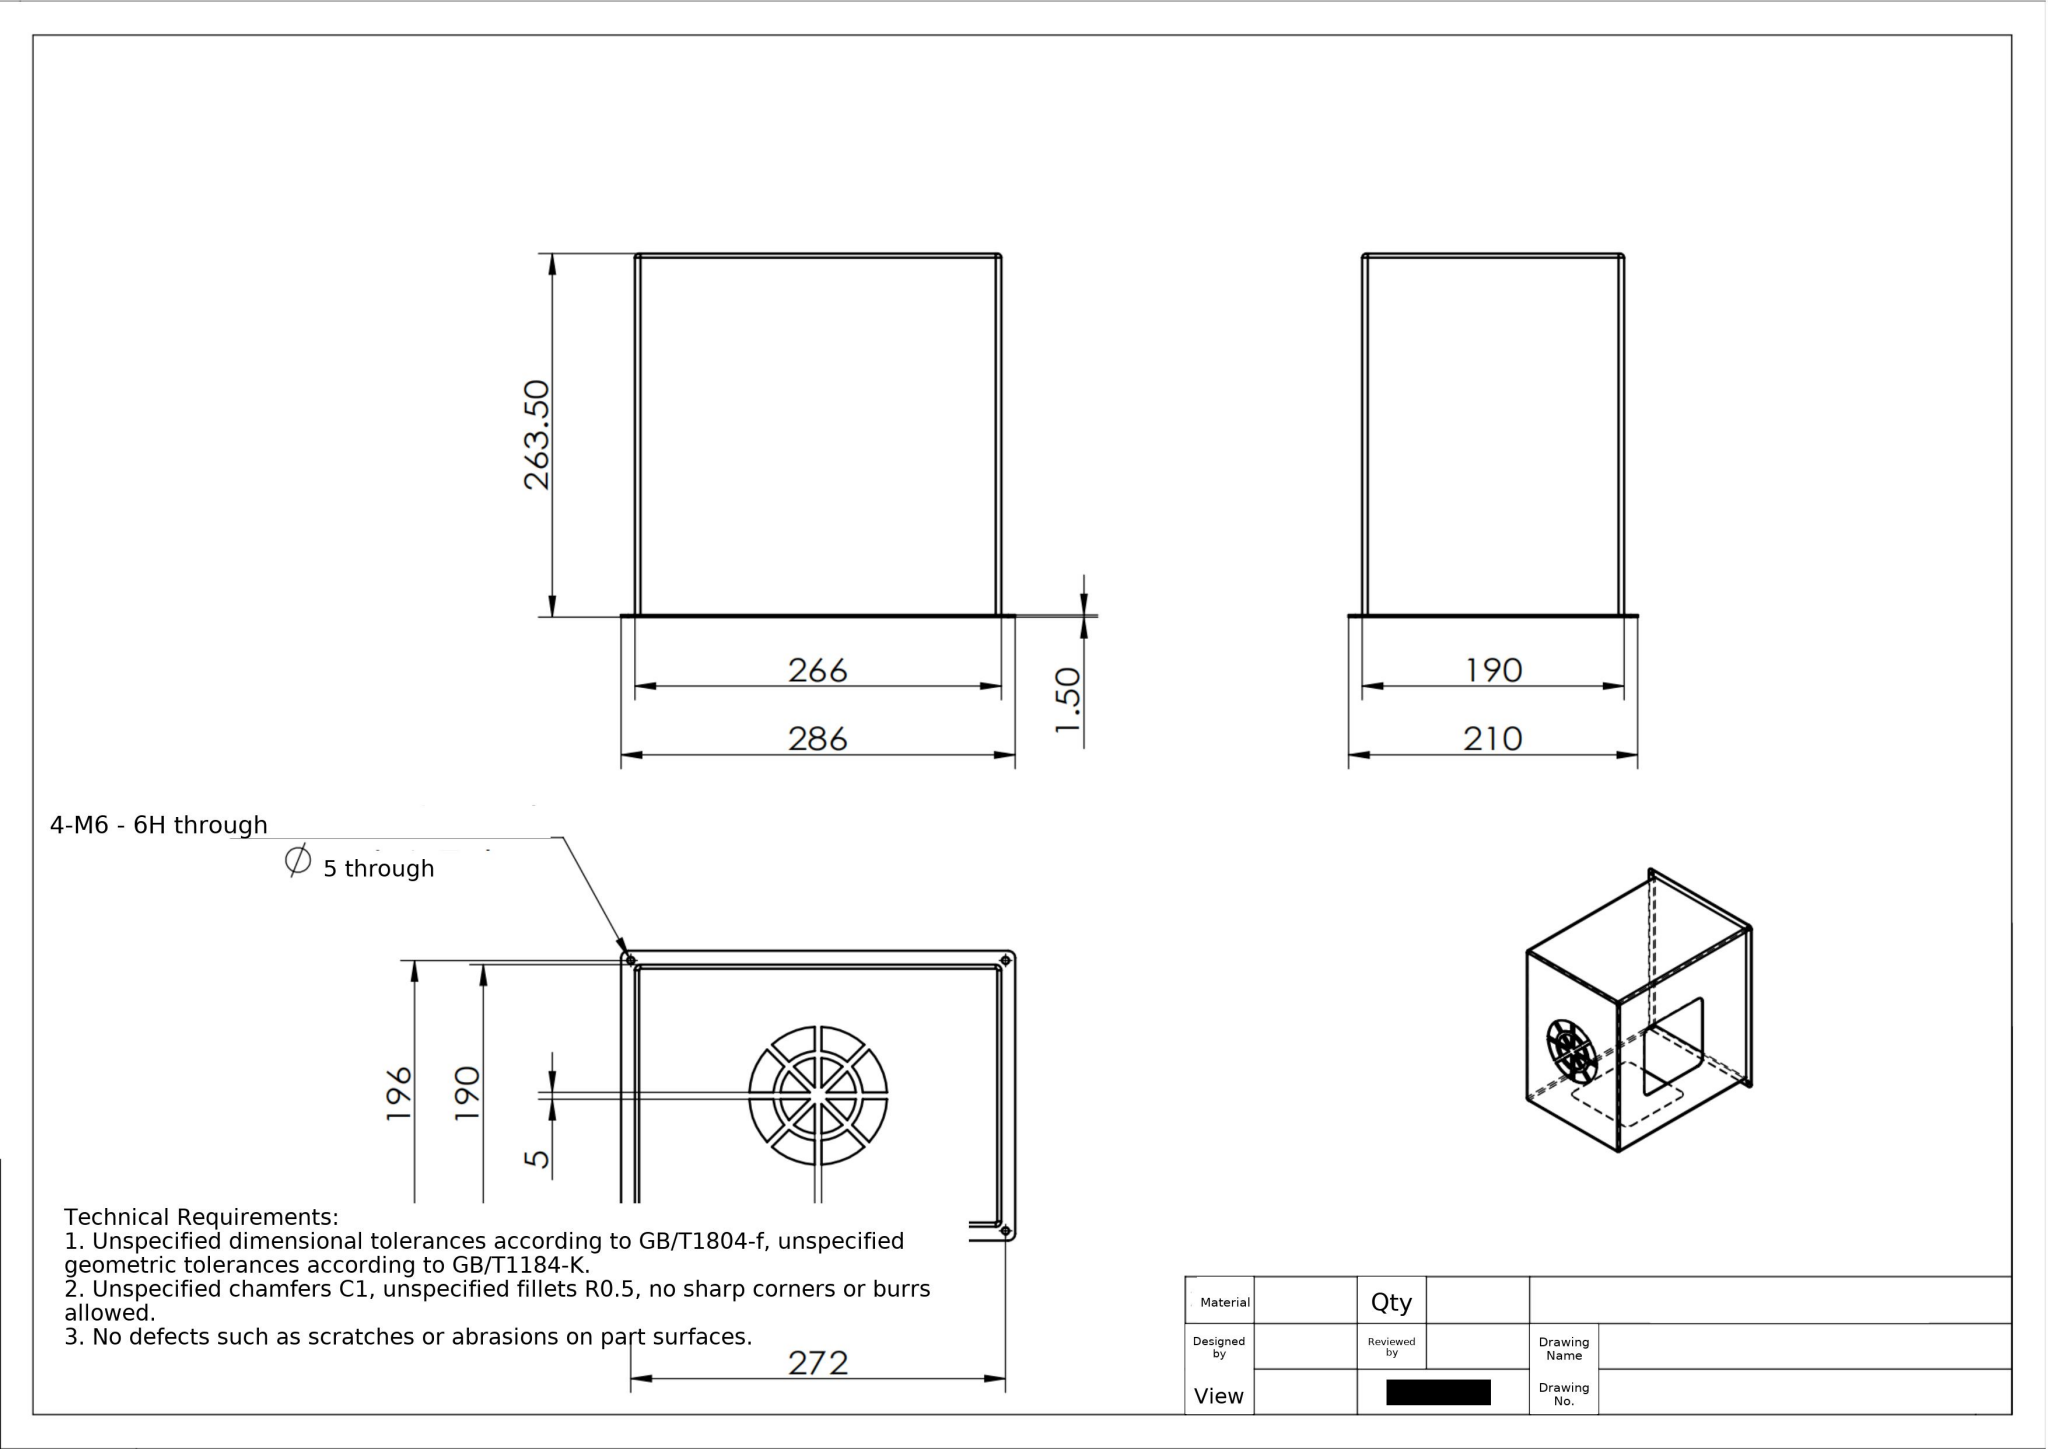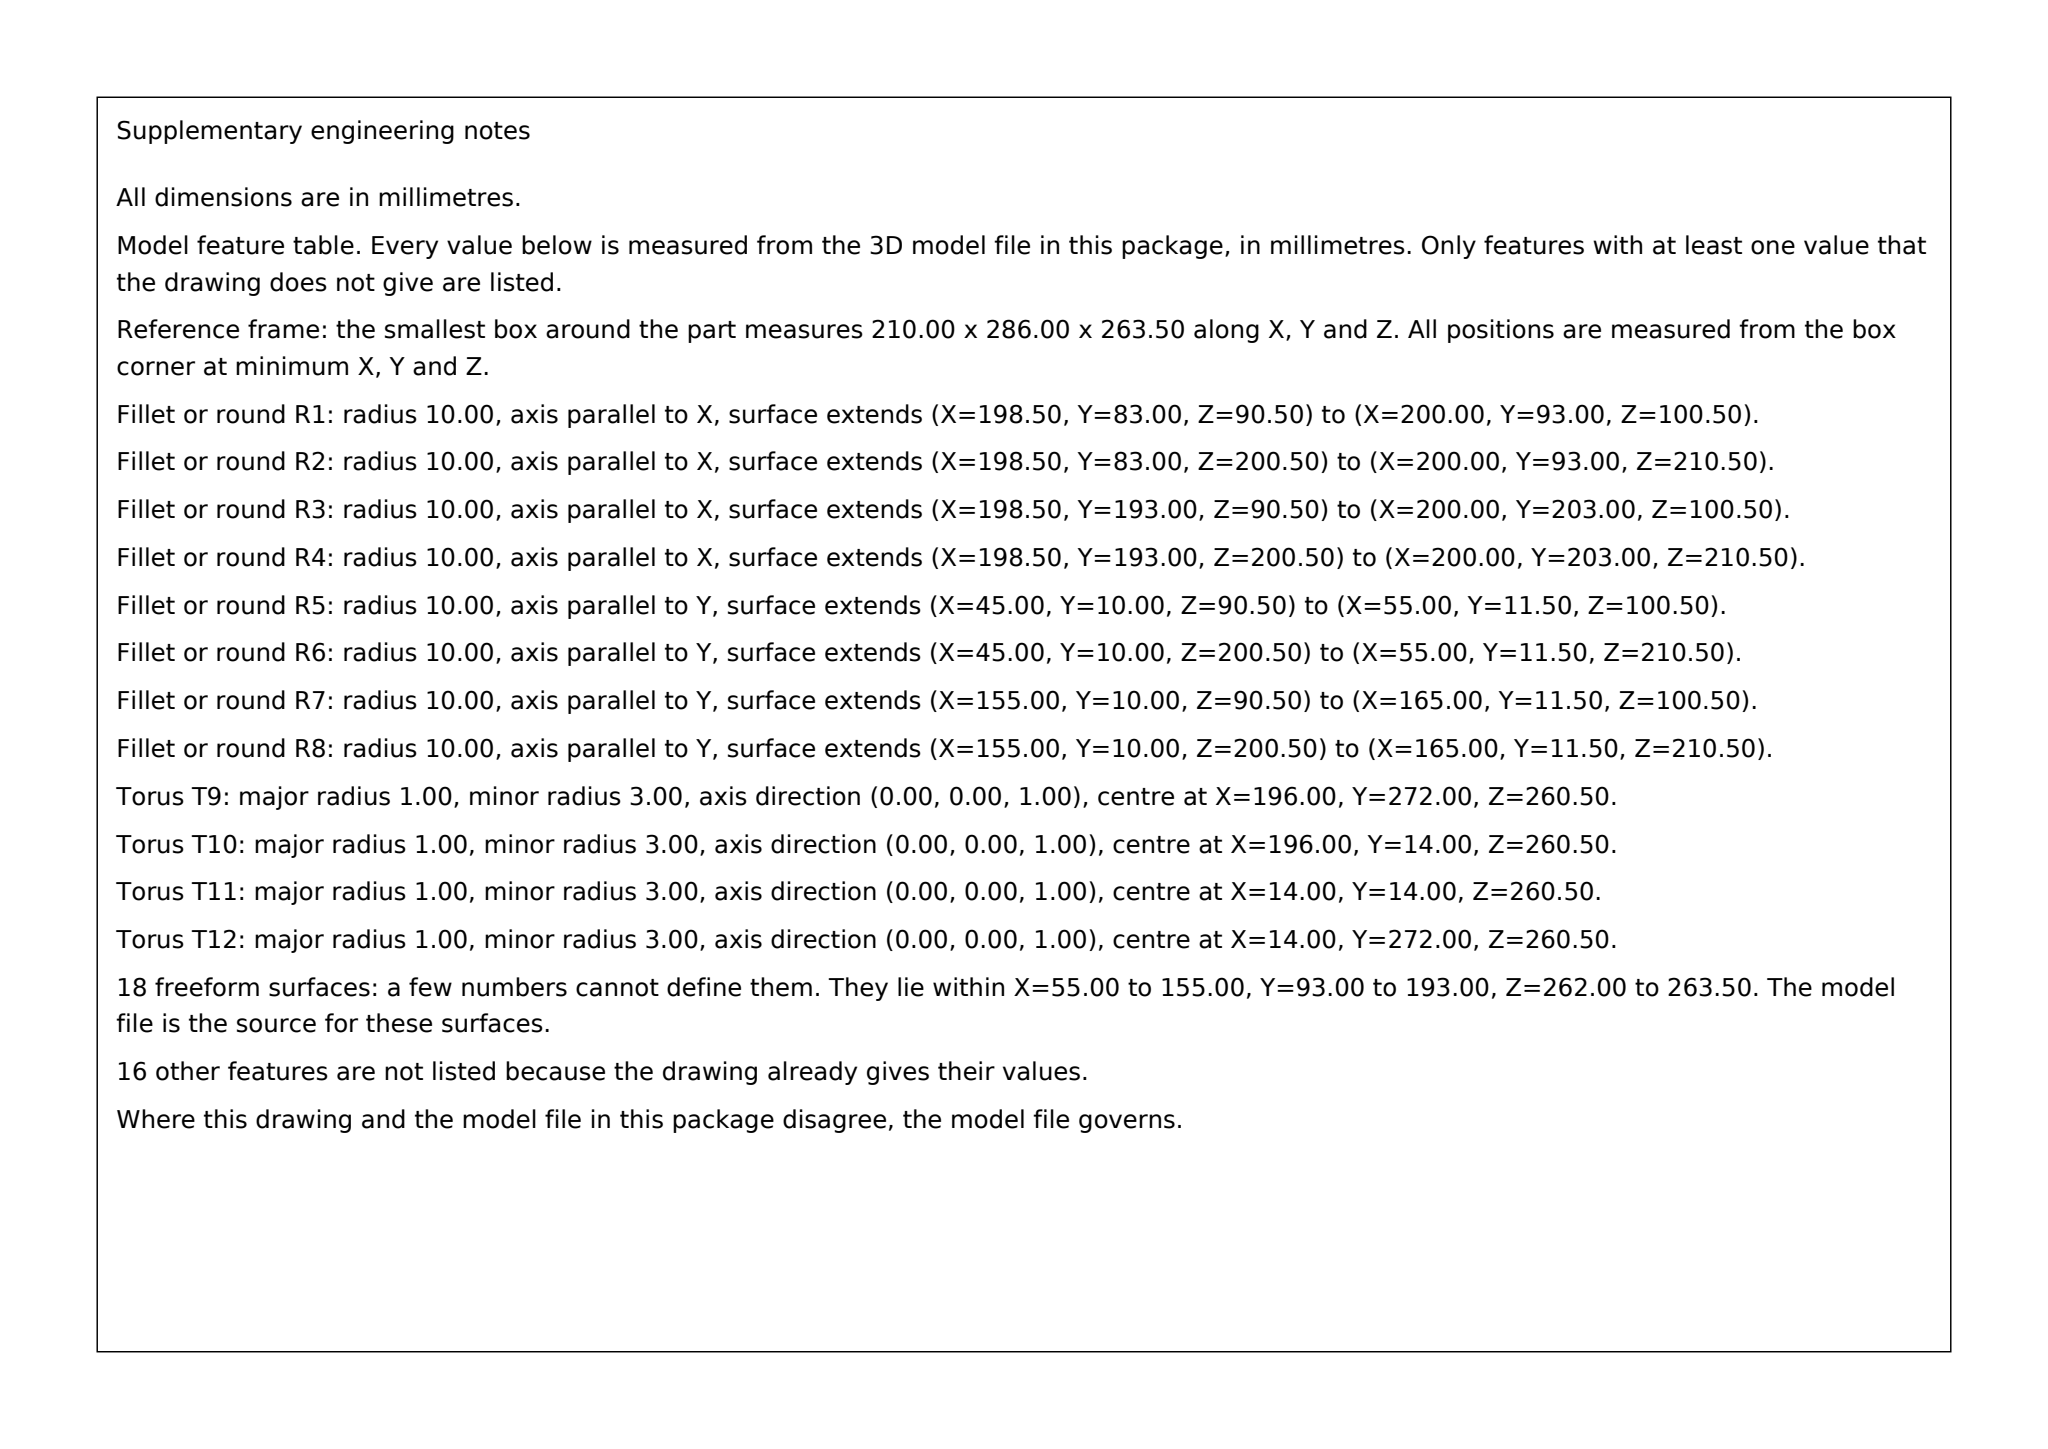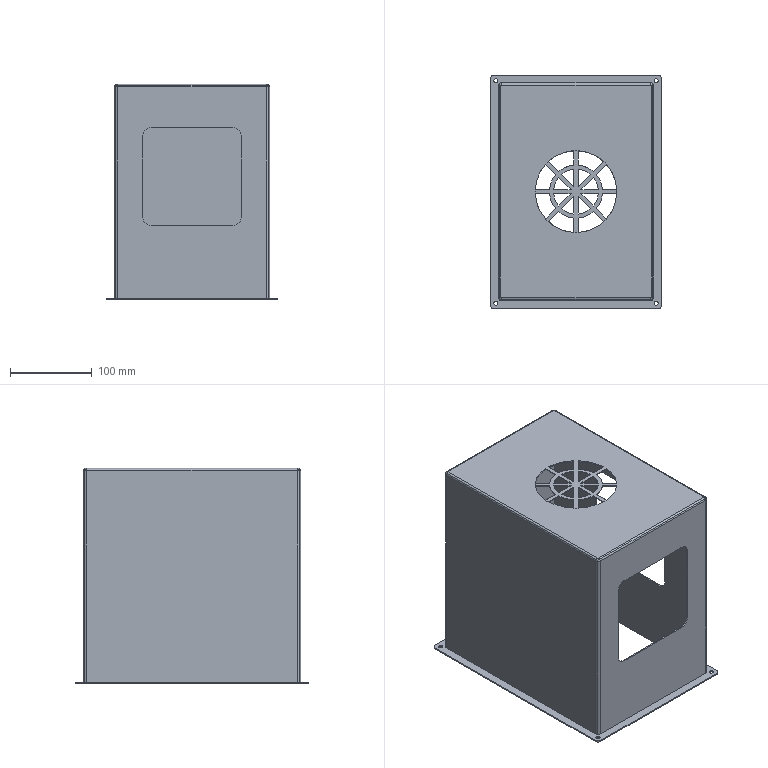Part | SolidWorks | mm | 1 solid | 107 faces | box 210 x 286 x 263.5 mm | volume 388558 mm3 | plane 57 | cylinder 28 | spline 18 | torus 4 | commonest cylinder face diameters 20 x8 5 x8 10 x4 8 x4 6 x4